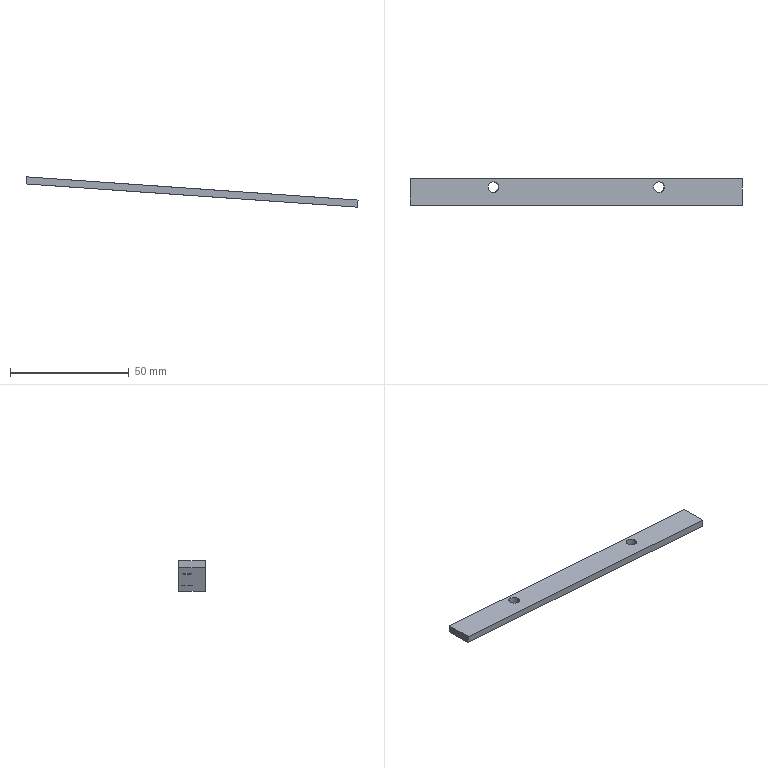Component | SolidWorks | FeedingPressureBlock-2 | 1 solid | 10 faces | box 139.87 x 11 x 12.76 mm | volume 4525 mm3 | plane 6 | cylinder 4 | commonest cylinder face diameters 4.5 x4
build123d program:
from build123d import *

# Parameters (mm, degrees)
SKETCH1_W           = 140
SKETCH1_H           = 11
BOSS_EXTRUDE1_DEPTH = 3
SKETCH2_R           = 2.25
CUT_EXTRUDE1_DEPTH  = 141.464


with BuildPart() as part:
    # Sketch1 → Boss-Extrude1 (new body)
    with BuildSketch(Plane.XY):
        with Locations((70, 5.5)):
            Rectangle(SKETCH1_W, SKETCH1_H)
    extrude(amount=BOSS_EXTRUDE1_DEPTH)

    # Sketch2 → Cut-Extrude1 (cut, through all)
    with BuildSketch(Plane.XY.offset(3)):
        with Locations((105, 3.5)):
            Circle(SKETCH2_R)
        with Locations((35, 3.5)):
            Circle(SKETCH2_R)
    extrude(amount=-CUT_EXTRUDE1_DEPTH, mode=Mode.SUBTRACT)


solid = part.part

# Placed as in the assembly
solid = solid.moved(Location((190.073, -233.176, 804.449), (-180, -4, 0)))
STEP:
#1=CARTESIAN_POINT('',(11.687,-9.318,31.259));
#2=VERTEX_POINT('',#1);
#3=CARTESIAN_POINT('',(11.51,-9.318,31.271));
#4=VERTEX_POINT('',#3);
#5=CARTESIAN_POINT('',(11.599,-9.318,31.265));
#6=DIRECTION('',(0.06976,-0.,0.9976));
#7=DIRECTION('',(-0.9976,0.,0.06976));
#8=AXIS2_PLACEMENT_3D('',#5,#6,#7);
#9=CIRCLE('',#8,0.08858);
#10=EDGE_CURVE('',#2,#4,#9,.T.);
#11=ORIENTED_EDGE('',*,*,#10,.F.);
#12=CARTESIAN_POINT('',(11.695,-9.318,31.377));
#13=VERTEX_POINT('',#12);
#14=CARTESIAN_POINT('',(11.687,-9.318,31.259));
#15=DIRECTION('',(0.06976,-0.,0.9976));
#16=VECTOR('',#15,39.37);
#17=LINE('',#14,#16);
#18=EDGE_CURVE('',#2,#13,#17,.T.);
#19=ORIENTED_EDGE('',*,*,#18,.T.);
#20=CARTESIAN_POINT('',(11.519,-9.318,31.389));
#21=VERTEX_POINT('',#20);
#22=CARTESIAN_POINT('',(11.607,-9.318,31.383));
#23=DIRECTION('',(0.06976,-0.,0.9976));
#24=DIRECTION('',(-0.9976,0.,0.06976));
#25=AXIS2_PLACEMENT_3D('',#22,#23,#24);
#26=CIRCLE('',#25,0.08858);
#27=EDGE_CURVE('',#13,#21,#26,.T.);
#28=ORIENTED_EDGE('',*,*,#27,.T.);
#29=CARTESIAN_POINT('',(11.51,-9.318,31.271));
#30=DIRECTION('',(0.06976,-0.,0.9976));
#31=VECTOR('',#30,39.37);
#32=LINE('',#29,#31);
#33=EDGE_CURVE('',#4,#21,#32,.T.);
#34=ORIENTED_EDGE('',*,*,#33,.F.);
#35=EDGE_LOOP('',(#11,#19,#28,#34));
#36=FACE_OUTER_BOUND('',#35,.T.);
#37=CARTESIAN_POINT('',(11.599,-9.318,31.265));
#38=DIRECTION('',(0.06976,-0.,0.9976));
#39=DIRECTION('',(-0.9976,0.,0.06976));
#40=AXIS2_PLACEMENT_3D('',#37,#38,#39);
#41=CYLINDRICAL_SURFACE('',#40,0.08858);
#42=ADVANCED_FACE('',(#36),#41,.F.);
#43=CARTESIAN_POINT('',(8.938,-9.318,31.451));
#44=VERTEX_POINT('',#43);
#45=CARTESIAN_POINT('',(8.761,-9.318,31.463));
#46=VERTEX_POINT('',#45);
#47=CARTESIAN_POINT('',(8.85,-9.318,31.457));
#48=DIRECTION('',(0.06976,-0.,0.9976));
#49=DIRECTION('',(-0.9976,0.,0.06976));
#50=AXIS2_PLACEMENT_3D('',#47,#48,#49);
#51=CIRCLE('',#50,0.08858);
#52=EDGE_CURVE('',#44,#46,#51,.T.);
#53=ORIENTED_EDGE('',*,*,#52,.F.);
#54=CARTESIAN_POINT('',(8.946,-9.318,31.569));
#55=VERTEX_POINT('',#54);
#56=CARTESIAN_POINT('',(8.938,-9.318,31.451));
#57=DIRECTION('',(0.06976,-0.,0.9976));
#58=VECTOR('',#57,39.37);
#59=LINE('',#56,#58);
#60=EDGE_CURVE('',#44,#55,#59,.T.);
#61=ORIENTED_EDGE('',*,*,#60,.T.);
#62=CARTESIAN_POINT('',(8.769,-9.318,31.581));
#63=VERTEX_POINT('',#62);
#64=CARTESIAN_POINT('',(8.858,-9.318,31.575));
#65=DIRECTION('',(0.06976,-0.,0.9976));
#66=DIRECTION('',(-0.9976,0.,0.06976));
#67=AXIS2_PLACEMENT_3D('',#64,#65,#66);
#68=CIRCLE('',#67,0.08858);
#69=EDGE_CURVE('',#55,#63,#68,.T.);
#70=ORIENTED_EDGE('',*,*,#69,.T.);
#71=CARTESIAN_POINT('',(8.761,-9.318,31.463));
#72=DIRECTION('',(0.06976,-0.,0.9976));
#73=VECTOR('',#72,39.37);
#74=LINE('',#71,#73);
#75=EDGE_CURVE('',#46,#63,#74,.T.);
#76=ORIENTED_EDGE('',*,*,#75,.F.);
#77=EDGE_LOOP('',(#53,#61,#70,#76));
#78=FACE_OUTER_BOUND('',#77,.T.);
#79=CARTESIAN_POINT('',(8.85,-9.318,31.457));
#80=DIRECTION('',(0.06976,-0.,0.9976));
#81=DIRECTION('',(-0.9976,0.,0.06976));
#82=AXIS2_PLACEMENT_3D('',#79,#80,#81);
#83=CYLINDRICAL_SURFACE('',#82,0.08858);
#84=ADVANCED_FACE('',(#78),#83,.F.);
#85=CARTESIAN_POINT('',(12.973,-9.613,31.169));
#86=VERTEX_POINT('',#85);
#87=CARTESIAN_POINT('',(12.973,-9.18,31.169));
#88=VERTEX_POINT('',#87);
#89=CARTESIAN_POINT('',(12.973,-9.18,31.169));
#90=DIRECTION('',(-0.,1.,0.));
#91=VECTOR('',#90,39.37);
#92=LINE('',#89,#91);
#93=EDGE_CURVE('',#86,#88,#92,.T.);
#94=ORIENTED_EDGE('',*,*,#93,.T.);
#95=CARTESIAN_POINT('',(12.982,-9.18,31.287));
#96=VERTEX_POINT('',#95);
#97=CARTESIAN_POINT('',(12.982,-9.18,31.287));
#98=DIRECTION('',(-0.06976,0.,-0.9976));
#99=VECTOR('',#98,39.37);
#100=LINE('',#97,#99);
#101=EDGE_CURVE('',#96,#88,#100,.T.);
#102=ORIENTED_EDGE('',*,*,#101,.F.);
#103=CARTESIAN_POINT('',(12.982,-9.613,31.287));
#104=VERTEX_POINT('',#103);
#105=CARTESIAN_POINT('',(12.982,-9.18,31.287));
#106=DIRECTION('',(-0.,1.,0.));
#107=VECTOR('',#106,39.37);
#108=LINE('',#105,#107);
#109=EDGE_CURVE('',#104,#96,#108,.T.);
#110=ORIENTED_EDGE('',*,*,#109,.F.);
#111=CARTESIAN_POINT('',(12.982,-9.613,31.287));
#112=DIRECTION('',(-0.06976,0.,-0.9976));
#113=VECTOR('',#112,39.37);
#114=LINE('',#111,#113);
#115=EDGE_CURVE('',#104,#86,#114,.T.);
#116=ORIENTED_EDGE('',*,*,#115,.T.);
#117=EDGE_LOOP('',(#94,#102,#110,#116));
#118=FACE_OUTER_BOUND('',#117,.T.);
#119=CARTESIAN_POINT('',(12.982,-9.18,31.287));
#120=DIRECTION('',(-0.9976,-0.,0.06976));
#121=DIRECTION('',(-0.06976,0.,-0.9976));
#122=AXIS2_PLACEMENT_3D('',#119,#120,#121);
#123=PLANE('',#122);
#124=ADVANCED_FACE('',(#118),#123,.F.);
#125=CARTESIAN_POINT('',(7.475,-9.18,31.553));
#126=VERTEX_POINT('',#125);
#127=CARTESIAN_POINT('',(12.973,-9.18,31.169));
#128=DIRECTION('',(-0.9976,-0.,0.06976));
#129=VECTOR('',#128,39.37);
#130=LINE('',#127,#129);
#131=EDGE_CURVE('',#88,#126,#130,.T.);
#132=ORIENTED_EDGE('',*,*,#131,.T.);
#133=CARTESIAN_POINT('',(7.483,-9.18,31.671));
#134=VERTEX_POINT('',#133);
#135=CARTESIAN_POINT('',(7.483,-9.18,31.671));
#136=DIRECTION('',(-0.06976,0.,-0.9976));
#137=VECTOR('',#136,39.37);
#138=LINE('',#135,#137);
#139=EDGE_CURVE('',#134,#126,#138,.T.);
#140=ORIENTED_EDGE('',*,*,#139,.F.);
#141=CARTESIAN_POINT('',(12.982,-9.18,31.287));
#142=DIRECTION('',(-0.9976,-0.,0.06976));
#143=VECTOR('',#142,39.37);
#144=LINE('',#141,#143);
#145=EDGE_CURVE('',#96,#134,#144,.T.);
#146=ORIENTED_EDGE('',*,*,#145,.F.);
#147=ORIENTED_EDGE('',*,*,#101,.T.);
#148=EDGE_LOOP('',(#132,#140,#146,#147));
#149=FACE_OUTER_BOUND('',#148,.T.);
#150=CARTESIAN_POINT('',(12.982,-9.18,31.287));
#151=DIRECTION('',(0.,-1.,-0.));
#152=DIRECTION('',(0.06976,-0.,0.9976));
#153=AXIS2_PLACEMENT_3D('',#150,#151,#152);
#154=PLANE('',#153);
#155=ADVANCED_FACE('',(#149),#154,.F.);
#156=CARTESIAN_POINT('',(7.475,-9.613,31.553));
#157=VERTEX_POINT('',#156);
#158=CARTESIAN_POINT('',(7.475,-9.18,31.553));
#159=DIRECTION('',(0.,-1.,-0.));
#160=VECTOR('',#159,39.37);
#161=LINE('',#158,#160);
#162=EDGE_CURVE('',#126,#157,#161,.T.);
#163=ORIENTED_EDGE('',*,*,#162,.T.);
#164=CARTESIAN_POINT('',(7.483,-9.613,31.671));
#165=VERTEX_POINT('',#164);
#166=CARTESIAN_POINT('',(7.483,-9.613,31.671));
#167=DIRECTION('',(-0.06976,0.,-0.9976));
#168=VECTOR('',#167,39.37);
#169=LINE('',#166,#168);
#170=EDGE_CURVE('',#165,#157,#169,.T.);
#171=ORIENTED_EDGE('',*,*,#170,.F.);
#172=CARTESIAN_POINT('',(7.483,-9.18,31.671));
#173=DIRECTION('',(0.,-1.,-0.));
#174=VECTOR('',#173,39.37);
#175=LINE('',#172,#174);
#176=EDGE_CURVE('',#134,#165,#175,.T.);
#177=ORIENTED_EDGE('',*,*,#176,.F.);
#178=ORIENTED_EDGE('',*,*,#139,.T.);
#179=EDGE_LOOP('',(#163,#171,#177,#178));
#180=FACE_OUTER_BOUND('',#179,.T.);
#181=CARTESIAN_POINT('',(7.483,-9.18,31.671));
#182=DIRECTION('',(0.9976,0.,-0.06976));
#183=DIRECTION('',(0.06976,-0.,0.9976));
#184=AXIS2_PLACEMENT_3D('',#181,#182,#183);
#185=PLANE('',#184);
#186=ADVANCED_FACE('',(#180),#185,.F.);
#187=CARTESIAN_POINT('',(12.973,-9.613,31.169));
#188=DIRECTION('',(0.9976,0.,-0.06976));
#189=VECTOR('',#188,39.37);
#190=LINE('',#187,#189);
#191=EDGE_CURVE('',#157,#86,#190,.T.);
#192=ORIENTED_EDGE('',*,*,#191,.T.);
#193=ORIENTED_EDGE('',*,*,#115,.F.);
#194=CARTESIAN_POINT('',(12.982,-9.613,31.287));
#195=DIRECTION('',(0.9976,0.,-0.06976));
#196=VECTOR('',#195,39.37);
#197=LINE('',#194,#196);
#198=EDGE_CURVE('',#165,#104,#197,.T.);
#199=ORIENTED_EDGE('',*,*,#198,.F.);
#200=ORIENTED_EDGE('',*,*,#170,.T.);
#201=EDGE_LOOP('',(#192,#193,#199,#200));
#202=FACE_OUTER_BOUND('',#201,.T.);
#203=CARTESIAN_POINT('',(12.982,-9.613,31.287));
#204=DIRECTION('',(-0.,1.,0.));
#205=DIRECTION('',(-0.06976,0.,-0.9976));
#206=AXIS2_PLACEMENT_3D('',#203,#204,#205);
#207=PLANE('',#206);
#208=ADVANCED_FACE('',(#202),#207,.F.);
#209=CARTESIAN_POINT('',(11.607,-9.318,31.383));
#210=DIRECTION('',(0.06976,-0.,0.9976));
#211=DIRECTION('',(-0.9976,0.,0.06976));
#212=AXIS2_PLACEMENT_3D('',#209,#210,#211);
#213=CIRCLE('',#212,0.08858);
#214=EDGE_CURVE('',#21,#13,#213,.T.);
#215=ORIENTED_EDGE('',*,*,#214,.F.);
#216=ORIENTED_EDGE('',*,*,#27,.F.);
#217=EDGE_LOOP('',(#215,#216));
#218=FACE_BOUND('',#217,.T.);
#219=CARTESIAN_POINT('',(8.858,-9.318,31.575));
#220=DIRECTION('',(0.06976,-0.,0.9976));
#221=DIRECTION('',(-0.9976,0.,0.06976));
#222=AXIS2_PLACEMENT_3D('',#219,#220,#221);
#223=CIRCLE('',#222,0.08858);
#224=EDGE_CURVE('',#63,#55,#223,.T.);
#225=ORIENTED_EDGE('',*,*,#224,.F.);
#226=ORIENTED_EDGE('',*,*,#69,.F.);
#227=EDGE_LOOP('',(#225,#226));
#228=FACE_BOUND('',#227,.T.);
#229=ORIENTED_EDGE('',*,*,#109,.T.);
#230=ORIENTED_EDGE('',*,*,#145,.T.);
#231=ORIENTED_EDGE('',*,*,#176,.T.);
#232=ORIENTED_EDGE('',*,*,#198,.T.);
#233=EDGE_LOOP('',(#229,#230,#231,#232));
#234=FACE_OUTER_BOUND('',#233,.T.);
#235=CARTESIAN_POINT('',(12.982,-9.18,31.287));
#236=DIRECTION('',(-0.06976,0.,-0.9976));
#237=DIRECTION('',(0.9976,0.,-0.06976));
#238=AXIS2_PLACEMENT_3D('',#235,#236,#237);
#239=PLANE('',#238);
#240=ADVANCED_FACE('',(#218,#228,#234),#239,.F.);
#241=CARTESIAN_POINT('',(11.599,-9.318,31.265));
#242=DIRECTION('',(0.06976,-0.,0.9976));
#243=DIRECTION('',(-0.9976,0.,0.06976));
#244=AXIS2_PLACEMENT_3D('',#241,#242,#243);
#245=CIRCLE('',#244,0.08858);
#246=EDGE_CURVE('',#4,#2,#245,.T.);
#247=ORIENTED_EDGE('',*,*,#246,.T.);
#248=ORIENTED_EDGE('',*,*,#10,.T.);
#249=EDGE_LOOP('',(#247,#248));
#250=FACE_BOUND('',#249,.T.);
#251=CARTESIAN_POINT('',(8.85,-9.318,31.457));
#252=DIRECTION('',(0.06976,-0.,0.9976));
#253=DIRECTION('',(-0.9976,0.,0.06976));
#254=AXIS2_PLACEMENT_3D('',#251,#252,#253);
#255=CIRCLE('',#254,0.08858);
#256=EDGE_CURVE('',#46,#44,#255,.T.);
#257=ORIENTED_EDGE('',*,*,#256,.T.);
#258=ORIENTED_EDGE('',*,*,#52,.T.);
#259=EDGE_LOOP('',(#257,#258));
#260=FACE_BOUND('',#259,.T.);
#261=ORIENTED_EDGE('',*,*,#93,.F.);
#262=ORIENTED_EDGE('',*,*,#191,.F.);
#263=ORIENTED_EDGE('',*,*,#162,.F.);
#264=ORIENTED_EDGE('',*,*,#131,.F.);
#265=EDGE_LOOP('',(#261,#262,#263,#264));
#266=FACE_OUTER_BOUND('',#265,.T.);
#267=CARTESIAN_POINT('',(12.973,-9.18,31.169));
#268=DIRECTION('',(-0.06976,0.,-0.9976));
#269=DIRECTION('',(0.9976,0.,-0.06976));
#270=AXIS2_PLACEMENT_3D('',#267,#268,#269);
#271=PLANE('',#270);
#272=ADVANCED_FACE('',(#250,#260,#266),#271,.T.);
#273=ORIENTED_EDGE('',*,*,#60,.F.);
#274=ORIENTED_EDGE('',*,*,#256,.F.);
#275=ORIENTED_EDGE('',*,*,#75,.T.);
#276=ORIENTED_EDGE('',*,*,#224,.T.);
#277=EDGE_LOOP('',(#273,#274,#275,#276));
#278=FACE_OUTER_BOUND('',#277,.T.);
#279=CARTESIAN_POINT('',(8.85,-9.318,31.457));
#280=DIRECTION('',(0.06976,-0.,0.9976));
#281=DIRECTION('',(-0.9976,0.,0.06976));
#282=AXIS2_PLACEMENT_3D('',#279,#280,#281);
#283=CYLINDRICAL_SURFACE('',#282,0.08858);
#284=ADVANCED_FACE('',(#278),#283,.F.);
#285=ORIENTED_EDGE('',*,*,#18,.F.);
#286=ORIENTED_EDGE('',*,*,#246,.F.);
#287=ORIENTED_EDGE('',*,*,#33,.T.);
#288=ORIENTED_EDGE('',*,*,#214,.T.);
#289=EDGE_LOOP('',(#285,#286,#287,#288));
#290=FACE_OUTER_BOUND('',#289,.T.);
#291=CARTESIAN_POINT('',(11.599,-9.318,31.265));
#292=DIRECTION('',(0.06976,-0.,0.9976));
#293=DIRECTION('',(-0.9976,0.,0.06976));
#294=AXIS2_PLACEMENT_3D('',#291,#292,#293);
#295=CYLINDRICAL_SURFACE('',#294,0.08858);
#296=ADVANCED_FACE('',(#290),#295,.F.);
#297=CLOSED_SHELL('',(#42,#84,#124,#155,#186,#208,#240,#272,#284,#296));
#298=MANIFOLD_SOLID_BREP('',#297);
#299=CARTESIAN_POINT('',(0.,0.,0.));
#300=DIRECTION('',(0.,0.,1.));
#301=DIRECTION('',(1.,0.,0.));
#302=AXIS2_PLACEMENT_3D('',#299,#300,#301);
#303=(LENGTH_UNIT()NAMED_UNIT(*)SI_UNIT($,.METRE.));
#304=LENGTH_MEASURE_WITH_UNIT(LENGTH_MEASURE(0.0254),#303);
#305=DIMENSIONAL_EXPONENTS(1.,0.,0.,0.,0.,0.,0.);
#306=(CONVERSION_BASED_UNIT('',#304)LENGTH_UNIT()NAMED_UNIT(#305));
#307=UNCERTAINTY_MEASURE_WITH_UNIT(LENGTH_MEASURE(0.00001),#306,'','');
#308=(NAMED_UNIT(*)PLANE_ANGLE_UNIT()SI_UNIT($,.RADIAN.));
#309=(NAMED_UNIT(*)SI_UNIT($,.STERADIAN.)SOLID_ANGLE_UNIT());
#310=(GEOMETRIC_REPRESENTATION_CONTEXT(3)GLOBAL_UNCERTAINTY_ASSIGNED_CONTEXT((#307))GLOBAL_UNIT_ASSIGNED_CONTEXT((#306,#308,#309))REPRESENTATION_CONTEXT('',''));
#311=ADVANCED_BREP_SHAPE_REPRESENTATION('',(#298,#302),#310);
#312=COLOUR_RGB('',0.7922,0.8196,0.9333);
#313=FILL_AREA_STYLE_COLOUR('',#312);
#314=FILL_AREA_STYLE('',(#313));
#315=SURFACE_STYLE_FILL_AREA(#314);
#316=SURFACE_SIDE_STYLE('',(#315));
#317=SURFACE_STYLE_USAGE(.BOTH.,#316);
#318=PRESENTATION_STYLE_ASSIGNMENT((#317));
#319=STYLED_ITEM('',(#318),#298);
#320=(LENGTH_UNIT()NAMED_UNIT(*)SI_UNIT($,.METRE.));
#321=LENGTH_MEASURE_WITH_UNIT(LENGTH_MEASURE(0.0254),#320);
#322=DIMENSIONAL_EXPONENTS(1.,0.,0.,0.,0.,0.,0.);
#323=(CONVERSION_BASED_UNIT('',#321)LENGTH_UNIT()NAMED_UNIT(#322));
#324=UNCERTAINTY_MEASURE_WITH_UNIT(LENGTH_MEASURE(0.00001),#323,'','');
#325=(NAMED_UNIT(*)PLANE_ANGLE_UNIT()SI_UNIT($,.RADIAN.));
#326=(NAMED_UNIT(*)SI_UNIT($,.STERADIAN.)SOLID_ANGLE_UNIT());
#327=(GEOMETRIC_REPRESENTATION_CONTEXT(3)GLOBAL_UNCERTAINTY_ASSIGNED_CONTEXT((#324))GLOBAL_UNIT_ASSIGNED_CONTEXT((#323,#325,#326))REPRESENTATION_CONTEXT('',''));
#328=MECHANICAL_DESIGN_GEOMETRIC_PRESENTATION_REPRESENTATION('',(#319),#327);
#329=PRESENTATION_LAYER_ASSIGNMENT('','',(#319));